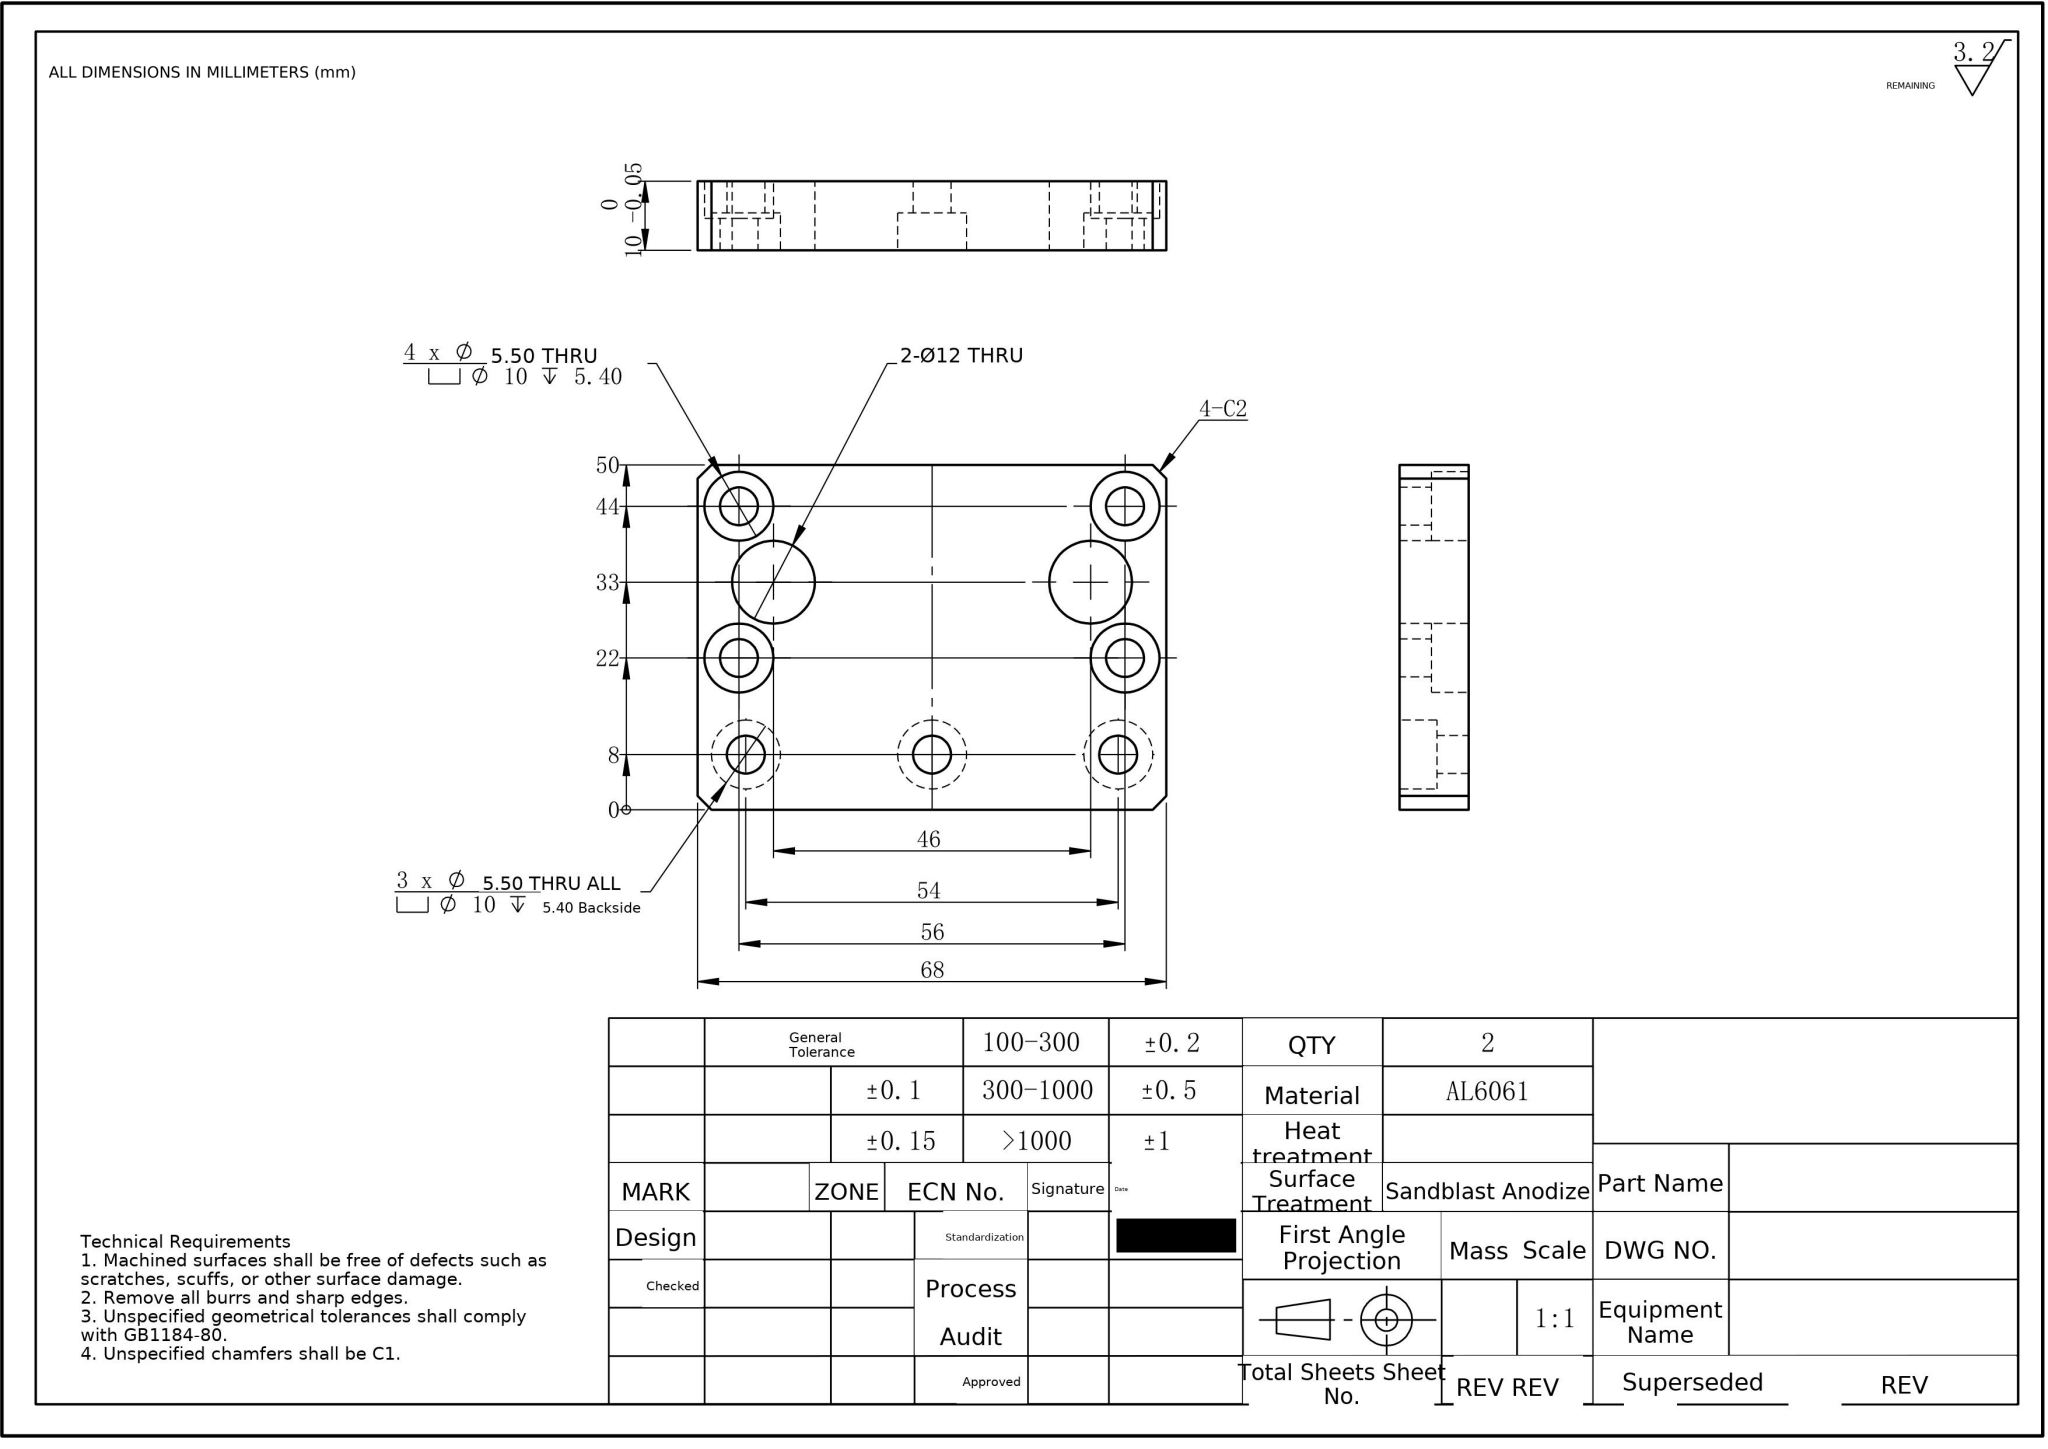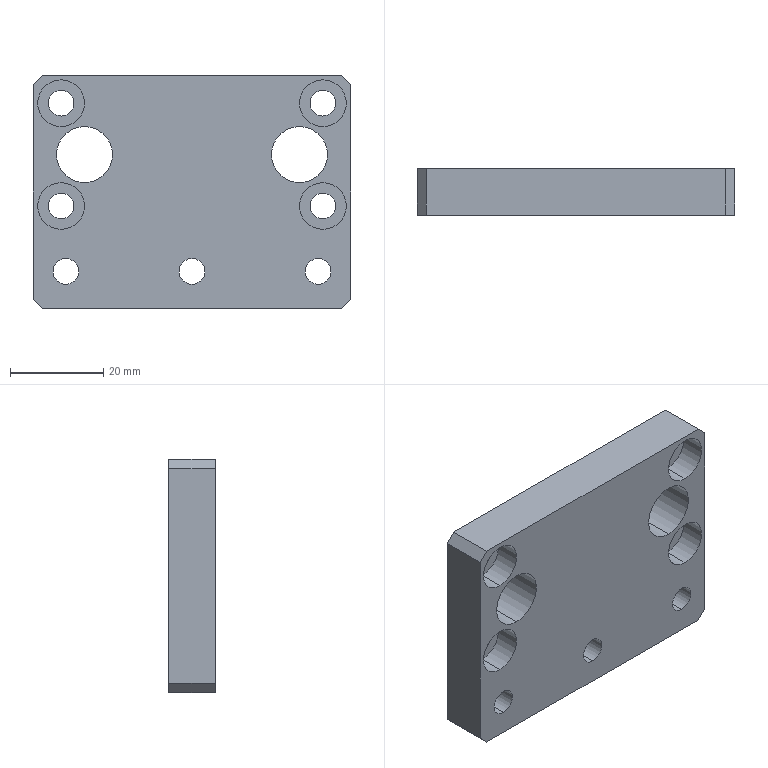Part | NX | mm | 1 solid | 49 faces | box 68 x 10 x 50 mm | volume 27924 mm3 | cylinder 32 | plane 17 | commonest cylinder face diameters 10 x14 5.5 x14 12 x4